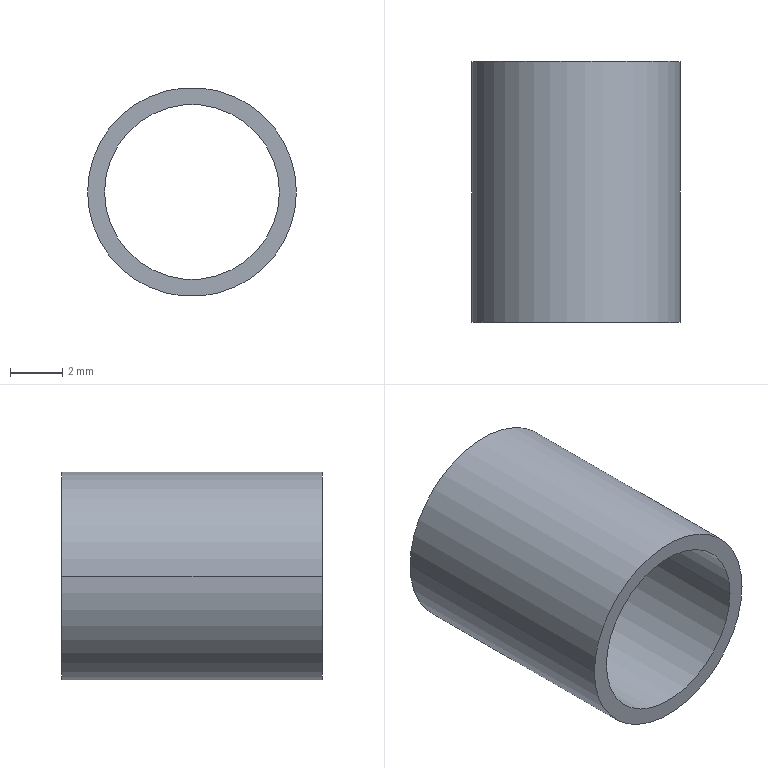Component | SolidWorks | YWL-D8-L10-3 | 1 solid | 6 faces | box 8 x 10 x 8 mm | volume 150 mm3 | cylinder 4 | plane 2 | commonest cylinder face diameters 6.7 x2 8 x2
build123d program:
from build123d import *

# Parameters (mm, degrees)
SKETCH1_R           = 4
SKETCH1_R_2         = 3.35
BOSS_EXTRUDE1_DEPTH = 10


with BuildPart() as part:
    # Sketch1 → Boss-Extrude1 (new body)
    with BuildSketch(Plane.XY):
        Circle(SKETCH1_R)
        Circle(SKETCH1_R_2, mode=Mode.SUBTRACT)
    extrude(amount=BOSS_EXTRUDE1_DEPTH)


solid = part.part

# Placed as in the assembly
solid = solid.moved(Location((-187.536, 73.25, 217.788), (90, 0, 0)))
STEP:
#1=COLOUR_RGB('',0.7922,0.8196,0.9333);
#2=FILL_AREA_STYLE_COLOUR('',#1);
#3=FILL_AREA_STYLE('',(#2));
#4=SURFACE_STYLE_FILL_AREA(#3);
#5=SURFACE_SIDE_STYLE('',(#4));
#6=SURFACE_STYLE_USAGE(.BOTH.,#5);
#7=PRESENTATION_STYLE_ASSIGNMENT((#6));
#8=CARTESIAN_POINT('',(-7.515,2.49,8.574));
#9=VERTEX_POINT('',#8);
#10=CARTESIAN_POINT('',(-7.251,2.49,8.574));
#11=VERTEX_POINT('',#10);
#12=CARTESIAN_POINT('',(-7.383,2.49,8.574));
#13=DIRECTION('',(-0.,-1.,0.));
#14=DIRECTION('',(1.,-0.,0.));
#15=AXIS2_PLACEMENT_3D('',#12,#13,#14);
#16=CIRCLE('',#15,0.1319);
#17=EDGE_CURVE('',#9,#11,#16,.T.);
#18=ORIENTED_EDGE('',*,*,#17,.T.);
#19=CARTESIAN_POINT('',(-7.251,2.884,8.574));
#20=VERTEX_POINT('',#19);
#21=CARTESIAN_POINT('',(-7.251,2.49,8.574));
#22=DIRECTION('',(0.,1.,-0.));
#23=VECTOR('',#22,39.37);
#24=LINE('',#21,#23);
#25=EDGE_CURVE('',#11,#20,#24,.T.);
#26=ORIENTED_EDGE('',*,*,#25,.T.);
#27=CARTESIAN_POINT('',(-7.515,2.884,8.574));
#28=VERTEX_POINT('',#27);
#29=CARTESIAN_POINT('',(-7.383,2.884,8.574));
#30=DIRECTION('',(-0.,-1.,0.));
#31=DIRECTION('',(1.,-0.,0.));
#32=AXIS2_PLACEMENT_3D('',#29,#30,#31);
#33=CIRCLE('',#32,0.1319);
#34=EDGE_CURVE('',#28,#20,#33,.T.);
#35=ORIENTED_EDGE('',*,*,#34,.F.);
#36=CARTESIAN_POINT('',(-7.515,2.49,8.574));
#37=DIRECTION('',(0.,1.,-0.));
#38=VECTOR('',#37,39.37);
#39=LINE('',#36,#38);
#40=EDGE_CURVE('',#9,#28,#39,.T.);
#41=ORIENTED_EDGE('',*,*,#40,.F.);
#42=EDGE_LOOP('',(#18,#26,#35,#41));
#43=FACE_OUTER_BOUND('',#42,.T.);
#44=CARTESIAN_POINT('',(-7.383,2.49,8.574));
#45=DIRECTION('',(0.,1.,-0.));
#46=DIRECTION('',(-1.,0.,-0.));
#47=AXIS2_PLACEMENT_3D('',#44,#45,#46);
#48=CYLINDRICAL_SURFACE('',#47,0.1319);
#49=ADVANCED_FACE('',(#43),#48,.F.);
#50=CARTESIAN_POINT('',(-7.226,2.49,8.574));
#51=VERTEX_POINT('',#50);
#52=CARTESIAN_POINT('',(-7.541,2.49,8.574));
#53=VERTEX_POINT('',#52);
#54=CARTESIAN_POINT('',(-7.383,2.49,8.574));
#55=DIRECTION('',(-0.,-1.,0.));
#56=DIRECTION('',(1.,-0.,0.));
#57=AXIS2_PLACEMENT_3D('',#54,#55,#56);
#58=CIRCLE('',#57,0.1575);
#59=EDGE_CURVE('',#51,#53,#58,.T.);
#60=ORIENTED_EDGE('',*,*,#59,.F.);
#61=CARTESIAN_POINT('',(-7.226,2.884,8.574));
#62=VERTEX_POINT('',#61);
#63=CARTESIAN_POINT('',(-7.226,2.49,8.574));
#64=DIRECTION('',(0.,1.,-0.));
#65=VECTOR('',#64,39.37);
#66=LINE('',#63,#65);
#67=EDGE_CURVE('',#51,#62,#66,.T.);
#68=ORIENTED_EDGE('',*,*,#67,.T.);
#69=CARTESIAN_POINT('',(-7.541,2.884,8.574));
#70=VERTEX_POINT('',#69);
#71=CARTESIAN_POINT('',(-7.383,2.884,8.574));
#72=DIRECTION('',(-0.,-1.,0.));
#73=DIRECTION('',(1.,-0.,0.));
#74=AXIS2_PLACEMENT_3D('',#71,#72,#73);
#75=CIRCLE('',#74,0.1575);
#76=EDGE_CURVE('',#62,#70,#75,.T.);
#77=ORIENTED_EDGE('',*,*,#76,.T.);
#78=CARTESIAN_POINT('',(-7.541,2.49,8.574));
#79=DIRECTION('',(0.,1.,-0.));
#80=VECTOR('',#79,39.37);
#81=LINE('',#78,#80);
#82=EDGE_CURVE('',#53,#70,#81,.T.);
#83=ORIENTED_EDGE('',*,*,#82,.F.);
#84=EDGE_LOOP('',(#60,#68,#77,#83));
#85=FACE_OUTER_BOUND('',#84,.T.);
#86=CARTESIAN_POINT('',(-7.383,2.49,8.574));
#87=DIRECTION('',(0.,1.,-0.));
#88=DIRECTION('',(-1.,0.,-0.));
#89=AXIS2_PLACEMENT_3D('',#86,#87,#88);
#90=CYLINDRICAL_SURFACE('',#89,0.1575);
#91=ADVANCED_FACE('',(#85),#90,.T.);
#92=CARTESIAN_POINT('',(-7.383,2.49,8.574));
#93=DIRECTION('',(-0.,-1.,0.));
#94=DIRECTION('',(1.,-0.,0.));
#95=AXIS2_PLACEMENT_3D('',#92,#93,#94);
#96=CIRCLE('',#95,0.1575);
#97=EDGE_CURVE('',#53,#51,#96,.T.);
#98=ORIENTED_EDGE('',*,*,#97,.T.);
#99=ORIENTED_EDGE('',*,*,#59,.T.);
#100=EDGE_LOOP('',(#98,#99));
#101=FACE_OUTER_BOUND('',#100,.T.);
#102=ORIENTED_EDGE('',*,*,#17,.F.);
#103=CARTESIAN_POINT('',(-7.383,2.49,8.574));
#104=DIRECTION('',(-0.,-1.,0.));
#105=DIRECTION('',(1.,-0.,0.));
#106=AXIS2_PLACEMENT_3D('',#103,#104,#105);
#107=CIRCLE('',#106,0.1319);
#108=EDGE_CURVE('',#11,#9,#107,.T.);
#109=ORIENTED_EDGE('',*,*,#108,.F.);
#110=EDGE_LOOP('',(#102,#109));
#111=FACE_BOUND('',#110,.T.);
#112=CARTESIAN_POINT('',(-7.383,2.49,8.574));
#113=DIRECTION('',(-0.,-1.,0.));
#114=DIRECTION('',(1.,-0.,0.));
#115=AXIS2_PLACEMENT_3D('',#112,#113,#114);
#116=PLANE('',#115);
#117=ADVANCED_FACE('',(#101,#111),#116,.T.);
#118=CARTESIAN_POINT('',(-7.383,2.884,8.574));
#119=DIRECTION('',(-0.,-1.,0.));
#120=DIRECTION('',(1.,-0.,0.));
#121=AXIS2_PLACEMENT_3D('',#118,#119,#120);
#122=CIRCLE('',#121,0.1575);
#123=EDGE_CURVE('',#70,#62,#122,.T.);
#124=ORIENTED_EDGE('',*,*,#123,.F.);
#125=ORIENTED_EDGE('',*,*,#76,.F.);
#126=EDGE_LOOP('',(#124,#125));
#127=FACE_OUTER_BOUND('',#126,.T.);
#128=ORIENTED_EDGE('',*,*,#34,.T.);
#129=CARTESIAN_POINT('',(-7.383,2.884,8.574));
#130=DIRECTION('',(-0.,-1.,0.));
#131=DIRECTION('',(1.,-0.,0.));
#132=AXIS2_PLACEMENT_3D('',#129,#130,#131);
#133=CIRCLE('',#132,0.1319);
#134=EDGE_CURVE('',#20,#28,#133,.T.);
#135=ORIENTED_EDGE('',*,*,#134,.T.);
#136=EDGE_LOOP('',(#128,#135));
#137=FACE_BOUND('',#136,.T.);
#138=CARTESIAN_POINT('',(-7.383,2.884,8.574));
#139=DIRECTION('',(-0.,-1.,0.));
#140=DIRECTION('',(1.,-0.,0.));
#141=AXIS2_PLACEMENT_3D('',#138,#139,#140);
#142=PLANE('',#141);
#143=ADVANCED_FACE('',(#127,#137),#142,.F.);
#144=ORIENTED_EDGE('',*,*,#67,.F.);
#145=ORIENTED_EDGE('',*,*,#97,.F.);
#146=ORIENTED_EDGE('',*,*,#82,.T.);
#147=ORIENTED_EDGE('',*,*,#123,.T.);
#148=EDGE_LOOP('',(#144,#145,#146,#147));
#149=FACE_OUTER_BOUND('',#148,.T.);
#150=CARTESIAN_POINT('',(-7.383,2.49,8.574));
#151=DIRECTION('',(0.,1.,-0.));
#152=DIRECTION('',(-1.,0.,-0.));
#153=AXIS2_PLACEMENT_3D('',#150,#151,#152);
#154=CYLINDRICAL_SURFACE('',#153,0.1575);
#155=ADVANCED_FACE('',(#149),#154,.T.);
#156=ORIENTED_EDGE('',*,*,#25,.F.);
#157=ORIENTED_EDGE('',*,*,#108,.T.);
#158=ORIENTED_EDGE('',*,*,#40,.T.);
#159=ORIENTED_EDGE('',*,*,#134,.F.);
#160=EDGE_LOOP('',(#156,#157,#158,#159));
#161=FACE_OUTER_BOUND('',#160,.T.);
#162=CARTESIAN_POINT('',(-7.383,2.49,8.574));
#163=DIRECTION('',(0.,1.,-0.));
#164=DIRECTION('',(-1.,0.,-0.));
#165=AXIS2_PLACEMENT_3D('',#162,#163,#164);
#166=CYLINDRICAL_SURFACE('',#165,0.1319);
#167=ADVANCED_FACE('',(#161),#166,.F.);
#168=CLOSED_SHELL('',(#49,#91,#117,#143,#155,#167));
#169=MANIFOLD_SOLID_BREP('',#168);
#170=STYLED_ITEM('',(#7),#169);
#171=(LENGTH_UNIT()NAMED_UNIT(*)SI_UNIT($,.METRE.));
#172=LENGTH_MEASURE_WITH_UNIT(LENGTH_MEASURE(0.0254),#171);
#173=DIMENSIONAL_EXPONENTS(1.,0.,0.,0.,0.,0.,0.);
#174=(CONVERSION_BASED_UNIT('',#172)LENGTH_UNIT()NAMED_UNIT(#173));
#175=UNCERTAINTY_MEASURE_WITH_UNIT(LENGTH_MEASURE(0.00001),#174,'','');
#176=(NAMED_UNIT(*)PLANE_ANGLE_UNIT()SI_UNIT($,.RADIAN.));
#177=(NAMED_UNIT(*)SI_UNIT($,.STERADIAN.)SOLID_ANGLE_UNIT());
#178=(GEOMETRIC_REPRESENTATION_CONTEXT(3)GLOBAL_UNCERTAINTY_ASSIGNED_CONTEXT((#175))GLOBAL_UNIT_ASSIGNED_CONTEXT((#174,#176,#177))REPRESENTATION_CONTEXT('',''));
#179=MECHANICAL_DESIGN_GEOMETRIC_PRESENTATION_REPRESENTATION('',(#170),#178);
#180=CARTESIAN_POINT('',(0.,0.,0.));
#181=DIRECTION('',(0.,0.,1.));
#182=DIRECTION('',(1.,0.,0.));
#183=AXIS2_PLACEMENT_3D('',#180,#181,#182);
#184=(LENGTH_UNIT()NAMED_UNIT(*)SI_UNIT($,.METRE.));
#185=LENGTH_MEASURE_WITH_UNIT(LENGTH_MEASURE(0.0254),#184);
#186=DIMENSIONAL_EXPONENTS(1.,0.,0.,0.,0.,0.,0.);
#187=(CONVERSION_BASED_UNIT('',#185)LENGTH_UNIT()NAMED_UNIT(#186));
#188=UNCERTAINTY_MEASURE_WITH_UNIT(LENGTH_MEASURE(0.00001),#187,'','');
#189=(NAMED_UNIT(*)PLANE_ANGLE_UNIT()SI_UNIT($,.RADIAN.));
#190=(NAMED_UNIT(*)SI_UNIT($,.STERADIAN.)SOLID_ANGLE_UNIT());
#191=(GEOMETRIC_REPRESENTATION_CONTEXT(3)GLOBAL_UNCERTAINTY_ASSIGNED_CONTEXT((#188))GLOBAL_UNIT_ASSIGNED_CONTEXT((#187,#189,#190))REPRESENTATION_CONTEXT('',''));
#192=ADVANCED_BREP_SHAPE_REPRESENTATION('',(#169,#183),#191);
#193=PRESENTATION_LAYER_ASSIGNMENT('','',(#170));